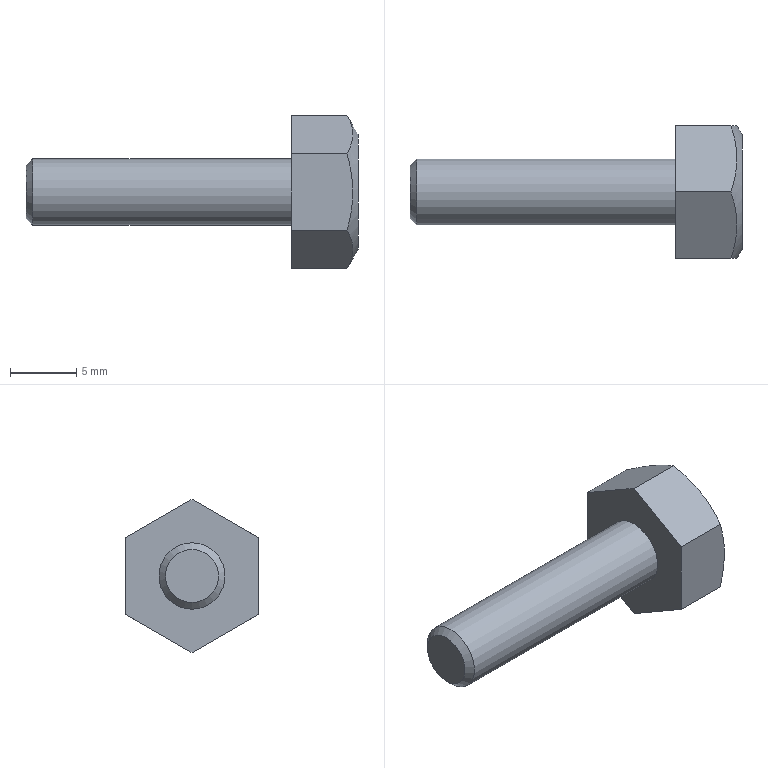Component | NX | SCREW_M5X20_2 | 1 solid | 12 faces | volume 816 mm3 | plane 9 | cone 2 | cylinder 1 | commonest cylinder face diameters 5 x1